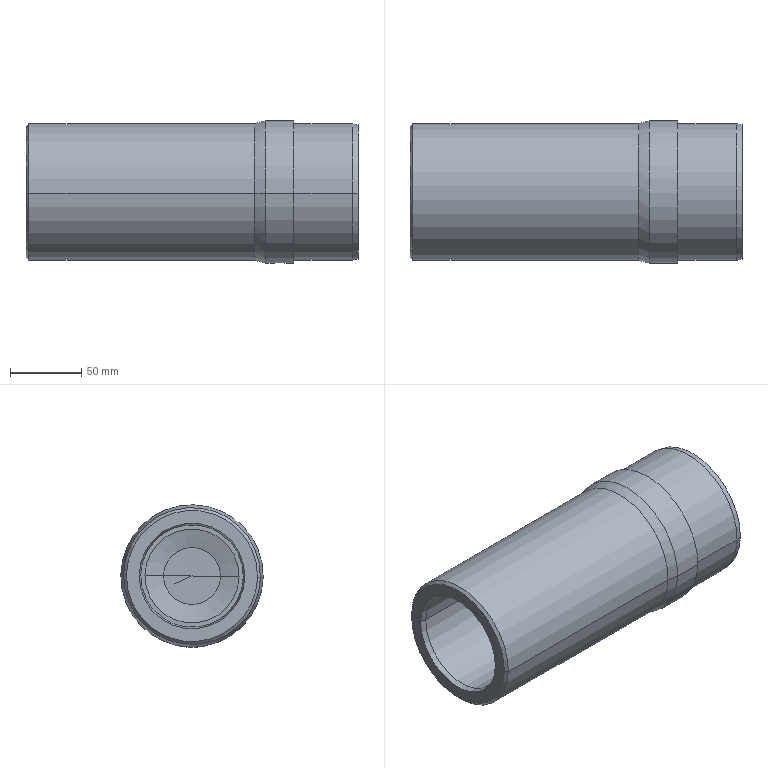Component | SolidWorks | 216InnerTubeAssembly-1_InnerTubeJoint-2 | 1 solid | 44 faces | box 233 x 100 x 100 mm | volume 1026015 mm3 | cylinder 21 | cone 16 | plane 7 | commonest cylinder face diameters 12 x5 40 x4 96 x4 66 x2 72 x2 100 x2 70 x2 | material Alloy Steel
build123d program:
from build123d import *

# Parameters (mm, degrees)
CUT_EXTRUDE1_REACH      = 245.581
CUT_EXTRUDE1_END_RADIUS = 50
SKETCH3_R               = 6
SKETCH1_W               = 0.1759
SKETCH1_H               = 3.3


with BuildPart() as part:
    # Model → Revolve1 (revolve)
    with BuildSketch(Plane.XY, mode=Mode.PRIVATE) as revolve1_sk:
        Polygon((-64.339, -0.1738), (-73.35, -0.1738), (-73.571, 19.826), (-86.571, 19.826), (-90.054, 32.826), (-173.054, 32.826), (-173.054, 35.826), (-229.054, 35.826), (-233.054, 36.898), (-233.054, 45.826), (-231.054, 47.826), (-72.519, 47.826), (-65.054, 49.826), (-45.054, 49.826), (-45.054, 47.826), (-4.065, 47.826), (-0.05449, 47.119), (-0.05449, 34.826), (-25.054, 34.826), (-24.875, 19.826), (-38.875, 19.826), (-38.875, 5.826), (-60.875, 5.826), align=None)
    revolve(revolve1_sk.sketch.rotate(Axis((-73.35, -0.1738, 0), (1, 0, 0)), 180), axis=Axis((-73.35, -0.1738, 0), (1, 0, 0)))

    # Cut-Extrude1: up to this cylinder (the profile starts inside it)
    cut_extrude1_end = Plane(origin=(-55.054, -0.1738, 0), z_dir=(-1, 0, 0)) * Cylinder(CUT_EXTRUDE1_END_RADIUS, 592.162, mode=Mode.PRIVATE)
    # Sketch3 → Cut-Extrude1 (cut, up to the surface)
    with BuildSketch(Plane.XY, mode=Mode.PRIVATE) as cut_extrude1_sk1:
        with Locations((-55.054, 0)):
            Circle(SKETCH3_R)
    cut_extrude1_tool1 = extrude(cut_extrude1_sk1.sketch, amount=-CUT_EXTRUDE1_REACH, mode=Mode.PRIVATE) & cut_extrude1_end
    add(cut_extrude1_tool1.solids().sort_by_distance((-55.054, 0, 0))[0], mode=Mode.SUBTRACT)

    # Sketch1 → Cut-Revolve1 (revolve, cut)
    with BuildSketch(Plane.XY, mode=Mode.PRIVATE) as cut_revolve1_sk:
        with Locations((-24.82, 20.976)):
            Rectangle(SKETCH1_W, SKETCH1_H)
    revolve(cut_revolve1_sk.sketch.rotate(Axis((-29.908, -0.1738, 0), (1, 0, 0)), 180), axis=Axis((-29.908, -0.1738, 0), (1, 0, 0)), mode=Mode.SUBTRACT)


solid = part.part

# Placed as in the assembly
solid = solid.moved(Location((1188.332, 0.1737, 0.003169), (1.033, 0, 0)))